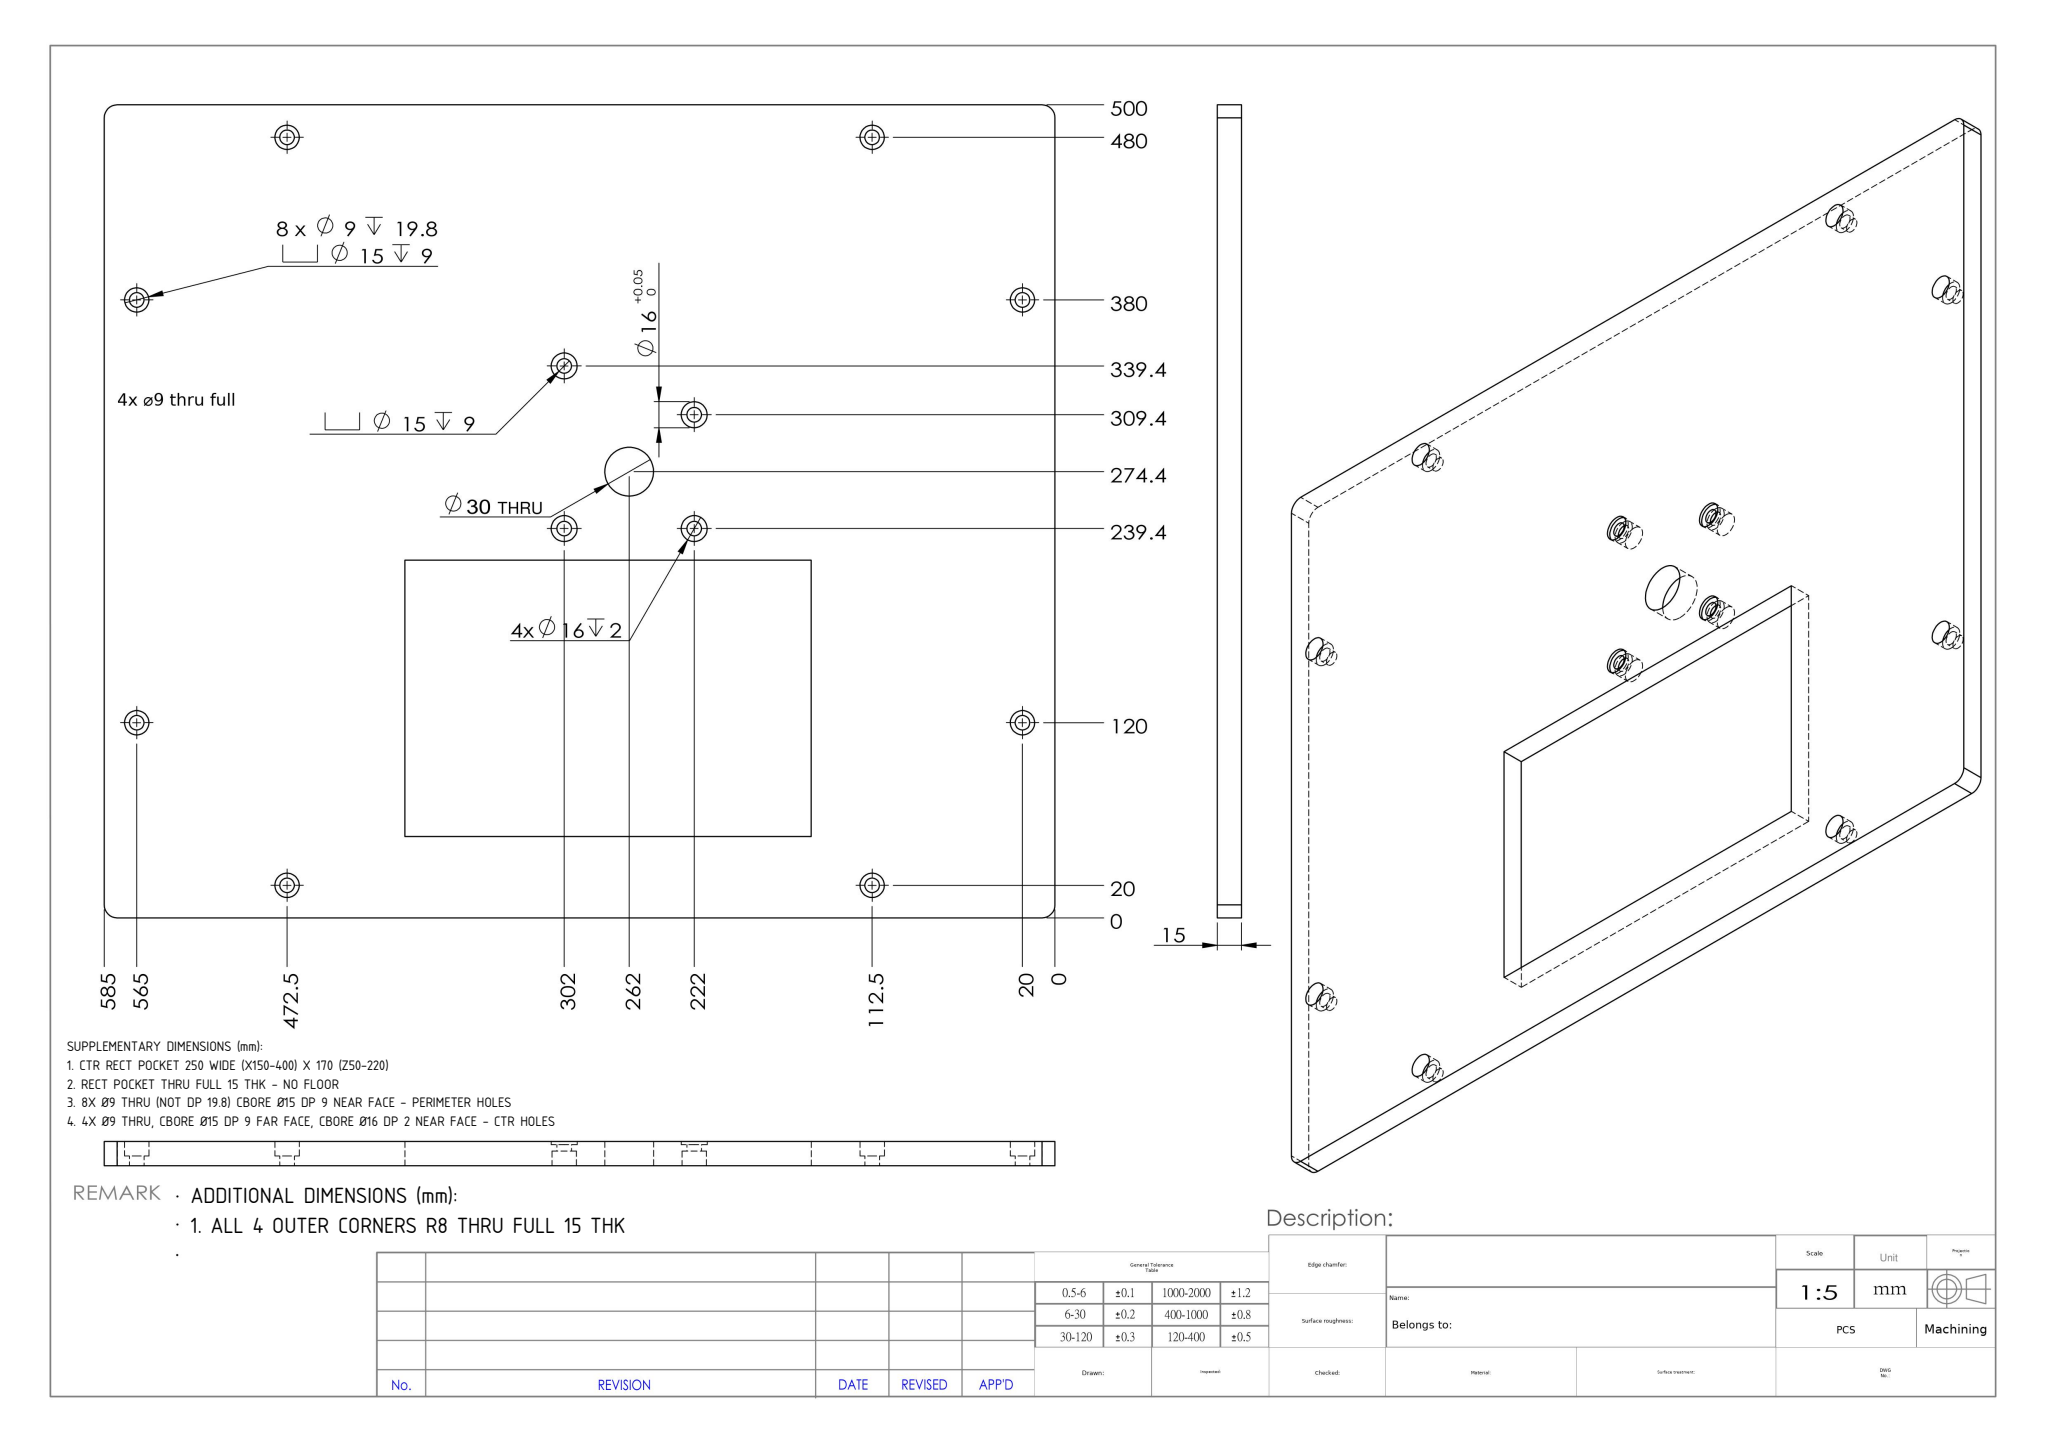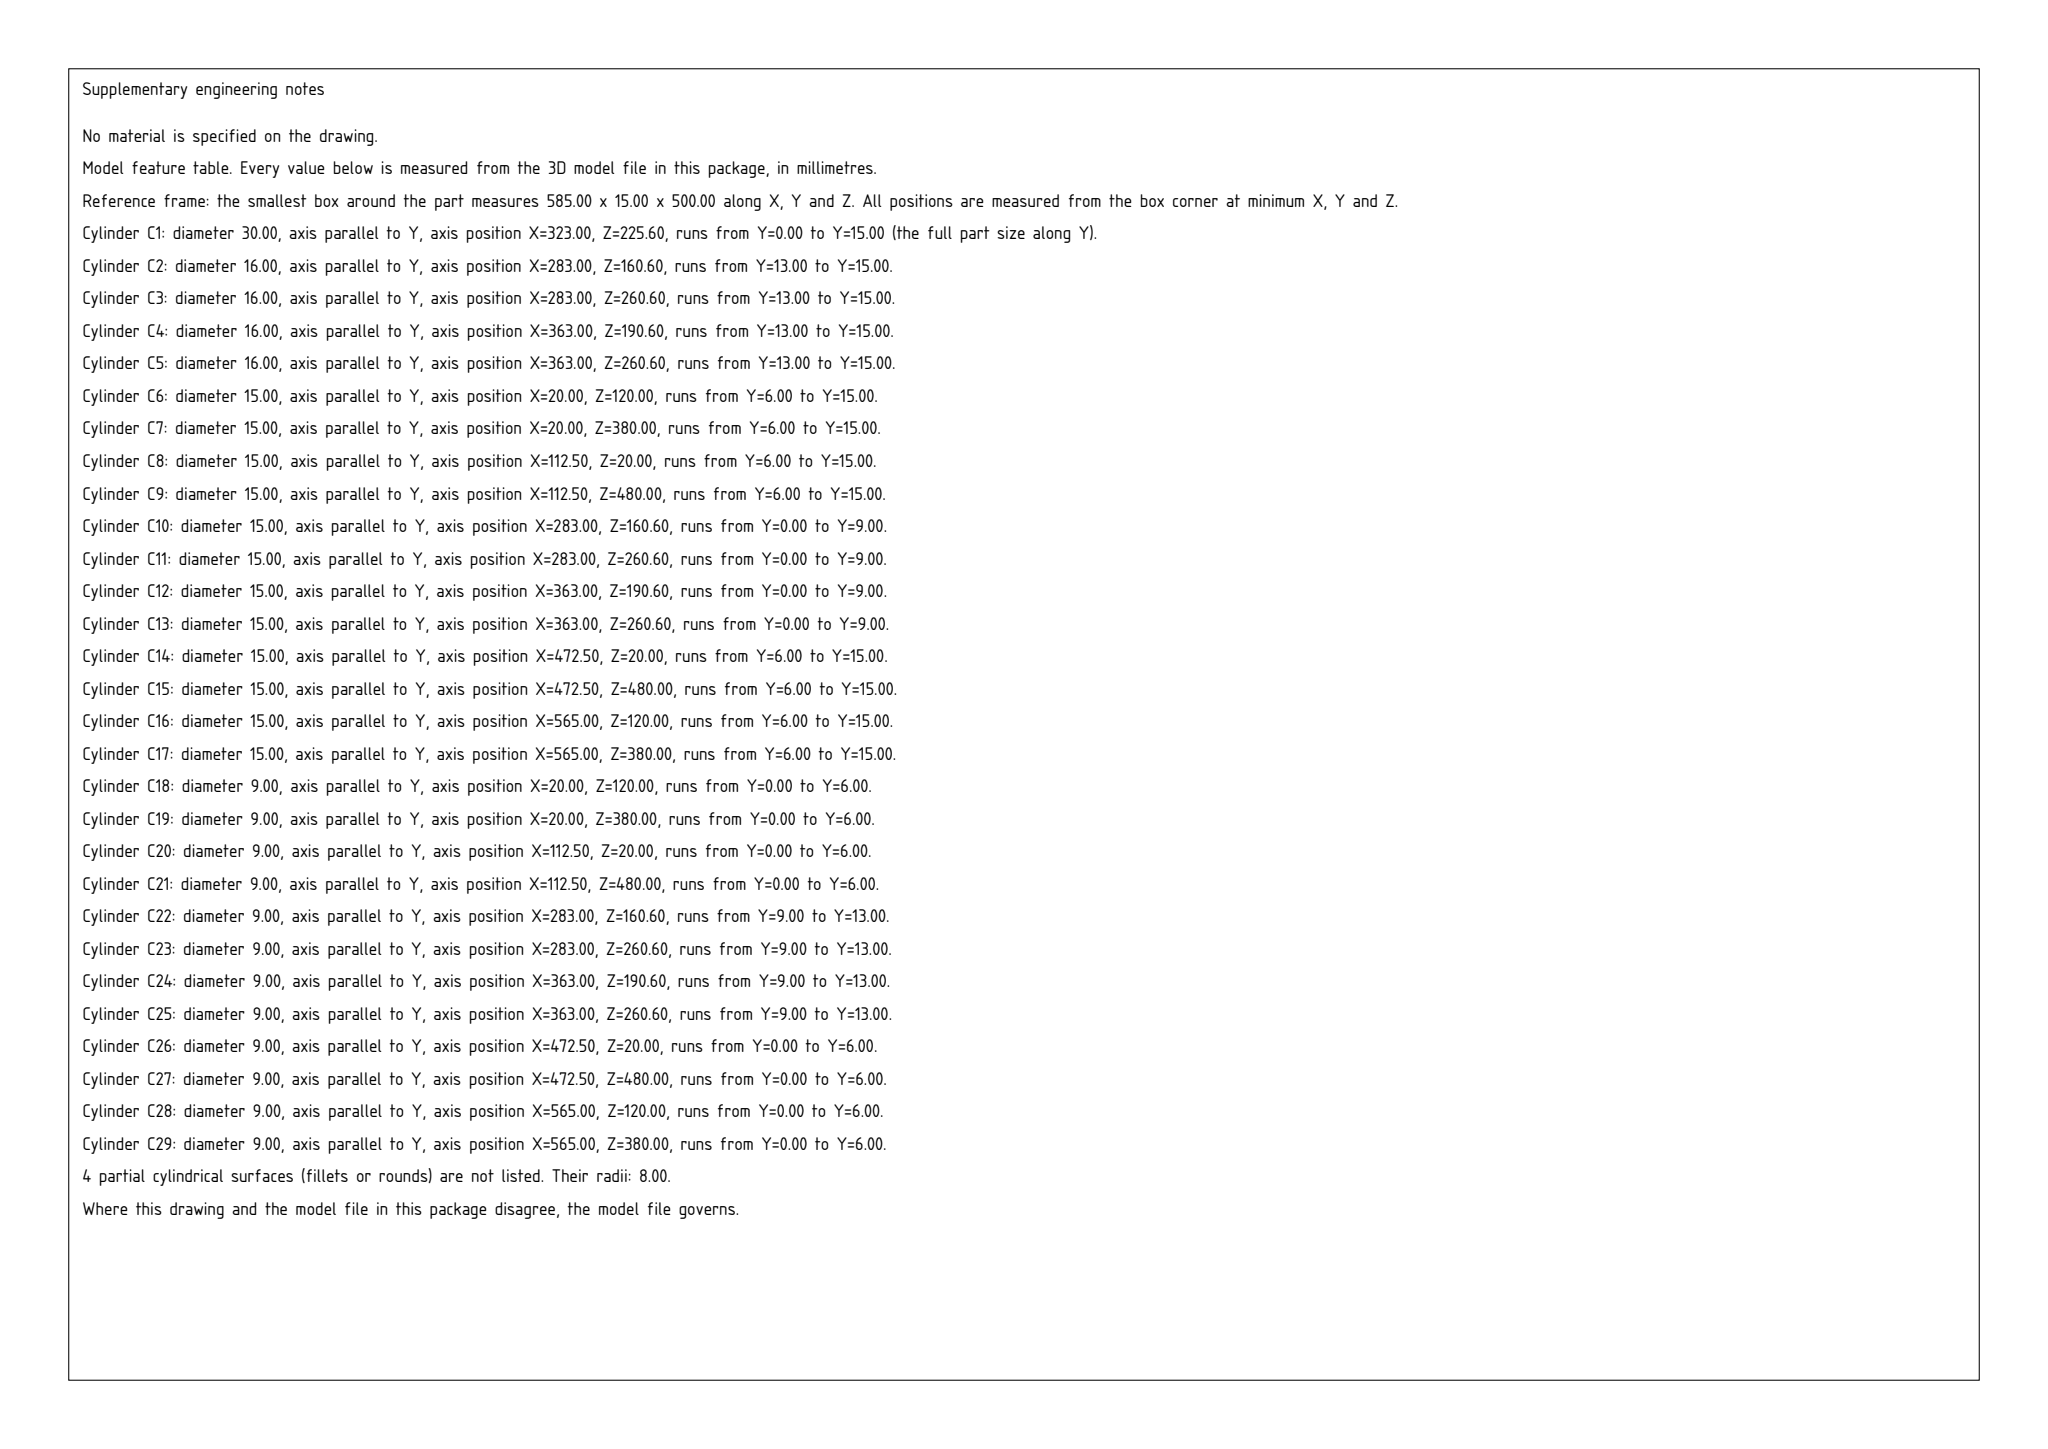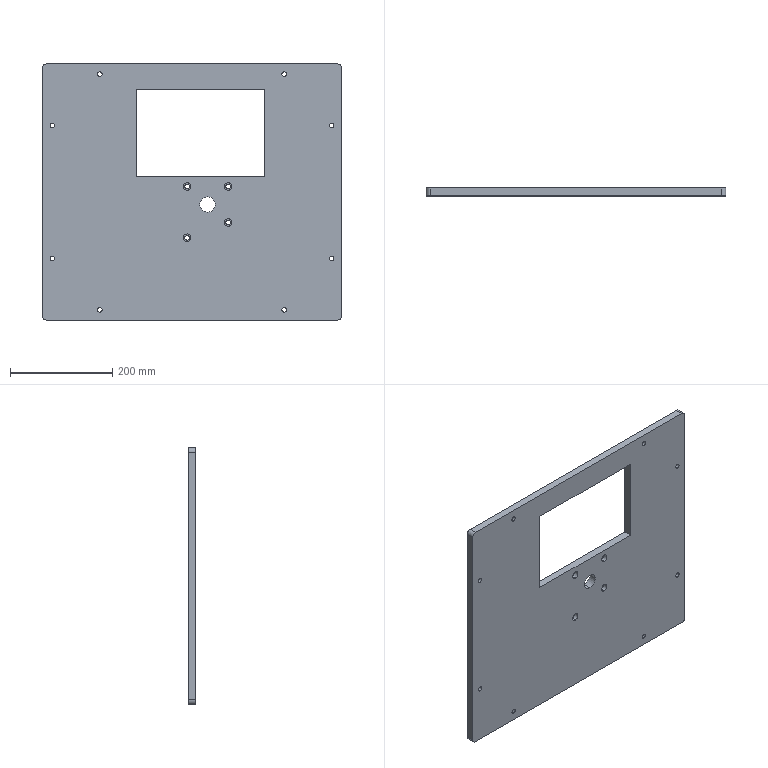Part | SolidWorks | mm | 1 solid | 88 faces | box 585 x 15 x 500 mm | volume 3714056 mm3 | cylinder 62 | plane 26 | commonest cylinder face diameters 15 x24 9 x24 16 x12 30 x2
build123d program:
from build123d import *

# Parameters (mm, degrees)
BOSS_EXTRUDE1_DEPTH                               = 15
BOSS_EXTRUDE1_DEPTH_BACK                          = 0.001
SKETCH1_W                                         = 585
SKETCH1_H                                         = 500
FILLET1_R                                         = 8
SKETCH2_R                                         = 8
CUT_EXTRUDE1_DEPTH                                = 2
HOLE_SIZE_ACCORDING_TO_HEXAGON_SOCKET_D           = 9
HOLE_SIZE_ACCORDING_TO_HEXAGON_SOCKET_DEPTH       = 19.8
HOLE_SIZE_ACCORDING_TO_HEXAGON_SOCKET_CBORE_D     = 15
HOLE_SIZE_ACCORDING_TO_HEXAGON_SOCKET_CBORE_DEPTH = 9
HOLE_SIZE_ACCORDING_TO_HEXAGON_SOCKET_TIP         = 2.704
SKETCH12_W                                        = 250
SKETCH12_H                                        = 170
CUT_EXTRUDE3_DEPTH                                = 386.073
HOLE_SIZE_ACCORDING_TO_HEXAGON_SO_2_D             = 9
HOLE_SIZE_ACCORDING_TO_HEXAGON_SO_2_CBORE_D       = 15
HOLE_SIZE_ACCORDING_TO_HEXAGON_SO_2_CBORE_DEPTH   = 9
SKETCH15_R                                        = 15
CUT_EXTRUDE4_DEPTH                                = 386.073


with BuildPart() as part:
    # Sketch1 → Boss-Extrude1 (new, two sides: drawn at the far end of the back side and taken through both)
    with BuildSketch(Plane(origin=(0, 0, 0), x_dir=(1, 0, 0), z_dir=(0, 1, 0)).offset(-BOSS_EXTRUDE1_DEPTH_BACK)):
        Rectangle(SKETCH1_W, SKETCH1_H)
    extrude(amount=BOSS_EXTRUDE1_DEPTH + BOSS_EXTRUDE1_DEPTH_BACK)

    # Fillet1
    fillet1_edges = [part.edges().sort_by_distance(p)[0] for p in [
        (292.5, 7.5, 250),
        (-292.5, 7.5, 250),
        (-292.5, 7.5, -250),
        (292.5, 7.5, -250),
    ]]
    fillet(fillet1_edges, radius=FILLET1_R)

    # Sketch2 → Cut-Extrude1 (cut)
    with BuildSketch(Plane(origin=(0, 15, 0), x_dir=(1, 0, 0), z_dir=(0, 1, 0))):
        with Locations(Location((70.5, 59.4, 0), (0, 0, 270))):
            Circle(SKETCH2_R)
        with Locations(Location((-9.5, 89.4, 0), (0, 0, 270))):
            Circle(SKETCH2_R)
        with Locations(Location((-9.5, -10.6, 0), (0, 0, 270))):
            Circle(SKETCH2_R)
        with Locations(Location((70.5, -10.6, 0), (0, 0, 270))):
            Circle(SKETCH2_R)
    extrude(amount=-CUT_EXTRUDE1_DEPTH, mode=Mode.SUBTRACT)

    # Hole Size _ according to_ Hexagon Socket
    with Locations(Plane(origin=(0, 15, 0), x_dir=(1, 0, 0), z_dir=(0, 1, 0))):
        with Locations((-272.5, 130), (-180, 230), (-272.5, -130), (180, 230), (180, -230), (-180, -230), (272.5, -130), (272.5, 130)):
            CounterBoreHole(HOLE_SIZE_ACCORDING_TO_HEXAGON_SOCKET_D / 2, HOLE_SIZE_ACCORDING_TO_HEXAGON_SOCKET_CBORE_D / 2, HOLE_SIZE_ACCORDING_TO_HEXAGON_SOCKET_CBORE_DEPTH, depth=HOLE_SIZE_ACCORDING_TO_HEXAGON_SOCKET_DEPTH)
            with Locations((0, 0, -(HOLE_SIZE_ACCORDING_TO_HEXAGON_SOCKET_DEPTH + HOLE_SIZE_ACCORDING_TO_HEXAGON_SOCKET_TIP / 2))):  # 118° drill point
                Cone(0, HOLE_SIZE_ACCORDING_TO_HEXAGON_SOCKET_D / 2, HOLE_SIZE_ACCORDING_TO_HEXAGON_SOCKET_TIP, mode=Mode.SUBTRACT)

    # Sketch12 → Cut-Extrude3 (cut, through all)
    with BuildSketch(Plane.XZ.offset(0.001)):
        with Locations((17.5, 115)):
            Rectangle(SKETCH12_W, SKETCH12_H)
    extrude(amount=-CUT_EXTRUDE3_DEPTH, mode=Mode.SUBTRACT)

    # Hole Size _ according to_ Hexagon So 2 (through all)
    with Locations(Plane(origin=(0, -0.001, 0), x_dir=(-1, 0, 0), z_dir=(0, -1, 0))):
        with Locations((9.5, -10.6), (-70.5, -10.6), (-70.5, 59.4), (9.5, 89.4)):
            CounterBoreHole(HOLE_SIZE_ACCORDING_TO_HEXAGON_SO_2_D / 2, HOLE_SIZE_ACCORDING_TO_HEXAGON_SO_2_CBORE_D / 2, HOLE_SIZE_ACCORDING_TO_HEXAGON_SO_2_CBORE_DEPTH)

    # Sketch15 → Cut-Extrude4 (cut, through all)
    with BuildSketch(Plane(origin=(0, 15, 0), x_dir=(1, 0, 0), z_dir=(0, 1, 0))):
        with Locations(Location((30.5, 24.4, 0), (0, 0, 270))):
            Circle(SKETCH15_R)
    extrude(amount=-CUT_EXTRUDE4_DEPTH, mode=Mode.SUBTRACT)


solid = part.part